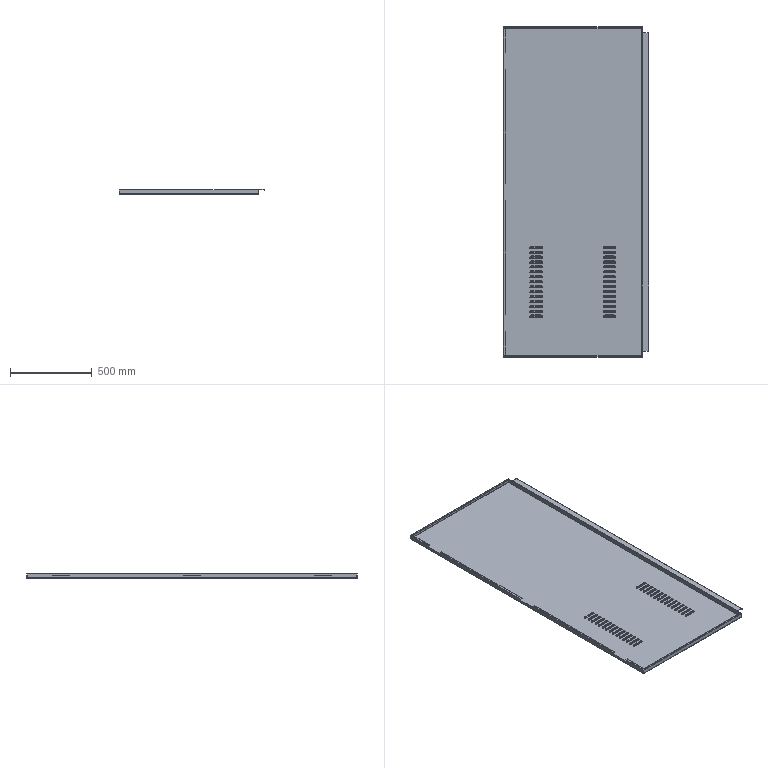Component | SolidWorks | SmallDoorPanel2-1 | 1 solid | 856 faces | volume 2969836 mm3 | cylinder 384 | torus 240 | plane 232 | commonest cylinder face diameters 8 x180 5 x90 11 x90 3.4 x12 0.4 x12